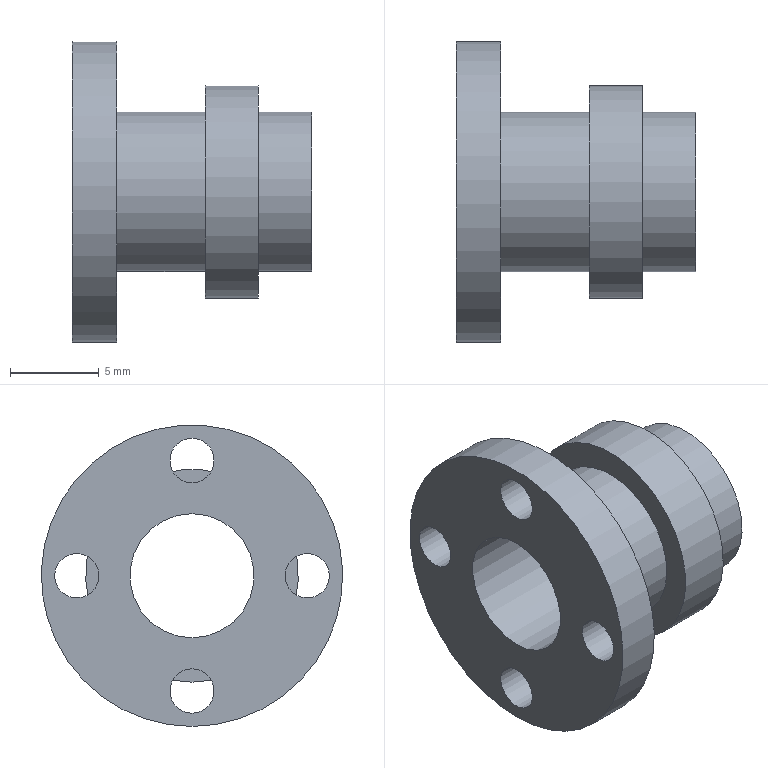Component | NX | EXT_CYLINDER_CONN_END_COVER | 1 solid | 14 faces | volume 847 mm3 | cylinder 9 | plane 5 | commonest cylinder face diameters 2.5 x4 9 x2 17 x1 12 x1 7 x1